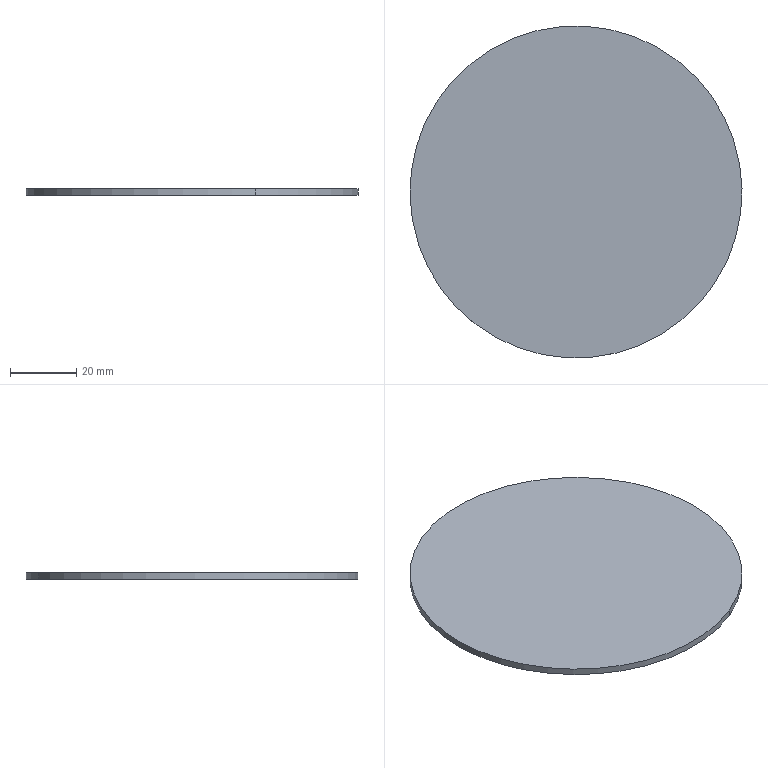Component | SolidWorks | BA850-01-02-01New-1 | 1 solid | 4 faces | box 100 x 100 x 2 mm | volume 15708 mm3 | cylinder 2 | plane 2 | commonest cylinder face diameters 100 x2 | material AISI 304
build123d program:
from build123d import *

# Parameters (mm, degrees)
SKETCH1_R           = 50
BOSS_EXTRUDE1_DEPTH = 2


with BuildPart() as part:
    # Sketch1 → Boss-Extrude1 (new body)
    with BuildSketch(Plane(origin=(0, 0, 0), x_dir=(1, 0, 0), z_dir=(0, 1, 0))):
        with Locations(Location((0, 0, 0), (0, 0, 270))):
            Circle(SKETCH1_R)
    extrude(amount=BOSS_EXTRUDE1_DEPTH)


solid = part.part

# Placed as in the assembly
solid = solid.moved(Location((1240.186, 993.812, 1434.454), (90, 0, 0)))
STEP:
#1=CARTESIAN_POINT('',(48.072,40.945,56.475));
#2=VERTEX_POINT('',#1);
#3=CARTESIAN_POINT('',(49.58,37.308,56.475));
#4=VERTEX_POINT('',#3);
#5=CARTESIAN_POINT('',(48.826,39.126,56.475));
#6=DIRECTION('',(0.,0.,-1.));
#7=DIRECTION('',(-0.383,0.9237,0.));
#8=AXIS2_PLACEMENT_3D('',#5,#6,#7);
#9=CIRCLE('',#8,1.969);
#10=EDGE_CURVE('',#2,#4,#9,.T.);
#11=ORIENTED_EDGE('',*,*,#10,.F.);
#12=CARTESIAN_POINT('',(48.072,40.945,56.553));
#13=VERTEX_POINT('',#12);
#14=CARTESIAN_POINT('',(48.072,40.945,56.475));
#15=DIRECTION('',(-0.,-0.,1.));
#16=VECTOR('',#15,39.37);
#17=LINE('',#14,#16);
#18=EDGE_CURVE('',#2,#13,#17,.T.);
#19=ORIENTED_EDGE('',*,*,#18,.T.);
#20=CARTESIAN_POINT('',(49.58,37.308,56.553));
#21=VERTEX_POINT('',#20);
#22=CARTESIAN_POINT('',(48.826,39.126,56.553));
#23=DIRECTION('',(0.,0.,-1.));
#24=DIRECTION('',(-0.383,0.9237,0.));
#25=AXIS2_PLACEMENT_3D('',#22,#23,#24);
#26=CIRCLE('',#25,1.969);
#27=EDGE_CURVE('',#13,#21,#26,.T.);
#28=ORIENTED_EDGE('',*,*,#27,.T.);
#29=CARTESIAN_POINT('',(49.58,37.308,56.475));
#30=DIRECTION('',(-0.,-0.,1.));
#31=VECTOR('',#30,39.37);
#32=LINE('',#29,#31);
#33=EDGE_CURVE('',#4,#21,#32,.T.);
#34=ORIENTED_EDGE('',*,*,#33,.F.);
#35=EDGE_LOOP('',(#11,#19,#28,#34));
#36=FACE_OUTER_BOUND('',#35,.T.);
#37=CARTESIAN_POINT('',(48.826,39.126,56.475));
#38=DIRECTION('',(-0.,-0.,1.));
#39=DIRECTION('',(0.383,-0.9237,-0.));
#40=AXIS2_PLACEMENT_3D('',#37,#38,#39);
#41=CYLINDRICAL_SURFACE('',#40,1.969);
#42=ADVANCED_FACE('',(#36),#41,.T.);
#43=ORIENTED_EDGE('',*,*,#18,.F.);
#44=CARTESIAN_POINT('',(48.826,39.126,56.475));
#45=DIRECTION('',(0.,0.,-1.));
#46=DIRECTION('',(-0.383,0.9237,0.));
#47=AXIS2_PLACEMENT_3D('',#44,#45,#46);
#48=CIRCLE('',#47,1.969);
#49=EDGE_CURVE('',#4,#2,#48,.T.);
#50=ORIENTED_EDGE('',*,*,#49,.F.);
#51=ORIENTED_EDGE('',*,*,#33,.T.);
#52=CARTESIAN_POINT('',(48.826,39.126,56.553));
#53=DIRECTION('',(0.,0.,-1.));
#54=DIRECTION('',(-0.383,0.9237,0.));
#55=AXIS2_PLACEMENT_3D('',#52,#53,#54);
#56=CIRCLE('',#55,1.969);
#57=EDGE_CURVE('',#21,#13,#56,.T.);
#58=ORIENTED_EDGE('',*,*,#57,.T.);
#59=EDGE_LOOP('',(#43,#50,#51,#58));
#60=FACE_OUTER_BOUND('',#59,.T.);
#61=CARTESIAN_POINT('',(48.826,39.126,56.475));
#62=DIRECTION('',(-0.,-0.,1.));
#63=DIRECTION('',(0.383,-0.9237,-0.));
#64=AXIS2_PLACEMENT_3D('',#61,#62,#63);
#65=CYLINDRICAL_SURFACE('',#64,1.969);
#66=ADVANCED_FACE('',(#60),#65,.T.);
#67=ORIENTED_EDGE('',*,*,#49,.T.);
#68=ORIENTED_EDGE('',*,*,#10,.T.);
#69=EDGE_LOOP('',(#67,#68));
#70=FACE_OUTER_BOUND('',#69,.T.);
#71=CARTESIAN_POINT('',(48.826,39.126,56.475));
#72=DIRECTION('',(-0.,0.,-1.));
#73=DIRECTION('',(-0.383,0.9237,0.));
#74=AXIS2_PLACEMENT_3D('',#71,#72,#73);
#75=PLANE('',#74);
#76=ADVANCED_FACE('',(#70),#75,.T.);
#77=ORIENTED_EDGE('',*,*,#57,.F.);
#78=ORIENTED_EDGE('',*,*,#27,.F.);
#79=EDGE_LOOP('',(#77,#78));
#80=FACE_OUTER_BOUND('',#79,.T.);
#81=CARTESIAN_POINT('',(48.826,39.126,56.553));
#82=DIRECTION('',(-0.,0.,-1.));
#83=DIRECTION('',(-0.383,0.9237,0.));
#84=AXIS2_PLACEMENT_3D('',#81,#82,#83);
#85=PLANE('',#84);
#86=ADVANCED_FACE('',(#80),#85,.F.);
#87=CLOSED_SHELL('',(#42,#66,#76,#86));
#88=MANIFOLD_SOLID_BREP('',#87);
#89=CARTESIAN_POINT('',(0.,0.,0.));
#90=DIRECTION('',(0.,0.,1.));
#91=DIRECTION('',(1.,0.,0.));
#92=AXIS2_PLACEMENT_3D('',#89,#90,#91);
#93=(LENGTH_UNIT()NAMED_UNIT(*)SI_UNIT($,.METRE.));
#94=LENGTH_MEASURE_WITH_UNIT(LENGTH_MEASURE(0.0254),#93);
#95=DIMENSIONAL_EXPONENTS(1.,0.,0.,0.,0.,0.,0.);
#96=(CONVERSION_BASED_UNIT('',#94)LENGTH_UNIT()NAMED_UNIT(#95));
#97=UNCERTAINTY_MEASURE_WITH_UNIT(LENGTH_MEASURE(0.00001),#96,'','');
#98=(NAMED_UNIT(*)PLANE_ANGLE_UNIT()SI_UNIT($,.RADIAN.));
#99=(NAMED_UNIT(*)SI_UNIT($,.STERADIAN.)SOLID_ANGLE_UNIT());
#100=(GEOMETRIC_REPRESENTATION_CONTEXT(3)GLOBAL_UNCERTAINTY_ASSIGNED_CONTEXT((#97))GLOBAL_UNIT_ASSIGNED_CONTEXT((#96,#98,#99))REPRESENTATION_CONTEXT('',''));
#101=ADVANCED_BREP_SHAPE_REPRESENTATION('',(#88,#92),#100);
#102=COLOUR_RGB('',0.7922,0.8196,0.9333);
#103=FILL_AREA_STYLE_COLOUR('',#102);
#104=FILL_AREA_STYLE('',(#103));
#105=SURFACE_STYLE_FILL_AREA(#104);
#106=SURFACE_SIDE_STYLE('',(#105));
#107=SURFACE_STYLE_USAGE(.BOTH.,#106);
#108=PRESENTATION_STYLE_ASSIGNMENT((#107));
#109=STYLED_ITEM('',(#108),#88);
#110=PRESENTATION_LAYER_ASSIGNMENT('','',(#109));
#111=(LENGTH_UNIT()NAMED_UNIT(*)SI_UNIT($,.METRE.));
#112=LENGTH_MEASURE_WITH_UNIT(LENGTH_MEASURE(0.0254),#111);
#113=DIMENSIONAL_EXPONENTS(1.,0.,0.,0.,0.,0.,0.);
#114=(CONVERSION_BASED_UNIT('',#112)LENGTH_UNIT()NAMED_UNIT(#113));
#115=UNCERTAINTY_MEASURE_WITH_UNIT(LENGTH_MEASURE(0.00001),#114,'','');
#116=(NAMED_UNIT(*)PLANE_ANGLE_UNIT()SI_UNIT($,.RADIAN.));
#117=(NAMED_UNIT(*)SI_UNIT($,.STERADIAN.)SOLID_ANGLE_UNIT());
#118=(GEOMETRIC_REPRESENTATION_CONTEXT(3)GLOBAL_UNCERTAINTY_ASSIGNED_CONTEXT((#115))GLOBAL_UNIT_ASSIGNED_CONTEXT((#114,#116,#117))REPRESENTATION_CONTEXT('',''));
#119=MECHANICAL_DESIGN_GEOMETRIC_PRESENTATION_REPRESENTATION('',(#109),#118);